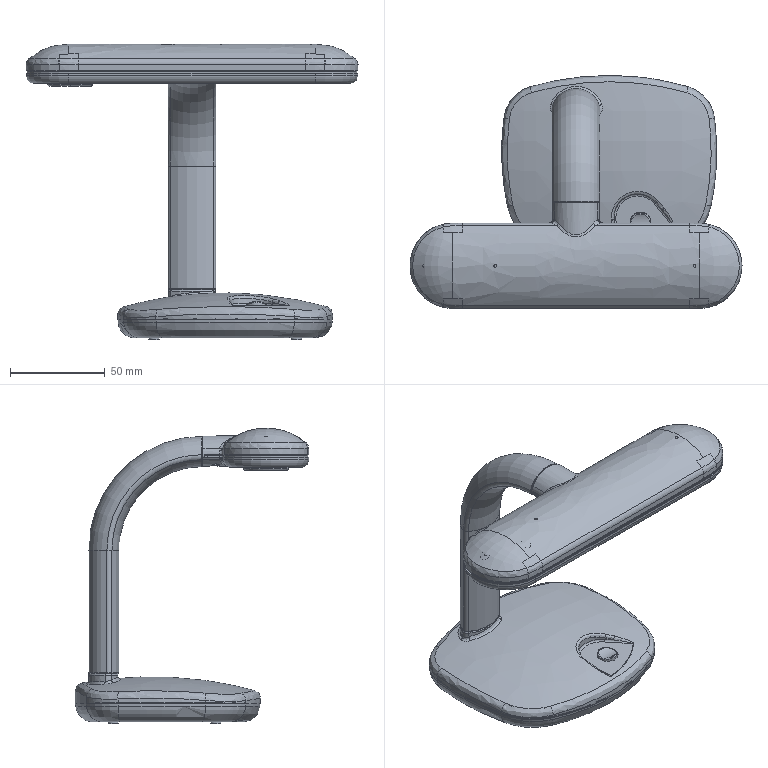Assembly | NX | mm | 9 component files | 9 solids | 848 faces | box 175 x 123.02 x 155.8 mm | volume 111281 mm3 | plane 324 | cylinder 252 | spline 133 | torus 67 | cone 66 | sphere 6 | commonest cylinder face diameters 1.5 x31 2 x25 5 x20 3 x20 1 x19 4 x18 6 x10 15 x8
Bill of materials:
unnamed part 1 | 1 |  | Flat rectangular plate with rounded corners and two through-holes, one near each end. Two rectangular tabs stick out from one long edge, leaving a notch between them.
unnamed part 2 | 1 |  | Flanged base with a short, slightly tapered cylindrical boss on top. The boss's top face is curved like a saddle. The flange has two lugs, each with a through-hole.
unnamed part 3 | 1 |  | Bent tubular body with a roughly 90-degree curve. It has a long straight leg ending in a smaller-diameter stepped end. A bore opens at the curved end.
unnamed part 4 | 1 |  | Elongated, pill-shaped low-profile body with a domed top. A short cylindrical stub sticks out sideways from the middle of one long side.
unnamed part 5 | 1 |  | Shallow, obround tray-like base with a perimeter rim. A raised rectangular block with one rounded end sits on the floor, small pins or bosses stand up from it, and a small bracket on one long side carries two holes.
unnamed part 6 | 1 |  | Rounded, squarish cover-like body with a gently domed top. It has two recessed pockets with through-holes: a small teardrop-shaped raised boss and a larger pocket shaped roughly like a sector.
unnamed part 7 | 1 |  | Bracket with a hexagonal outer profile and a rectangular through-opening. A flat mounting flange with two holed lugs extends from opposite sides, and there are also small holes in the side walls.
unnamed part 8 | 1 |  | Shallow open shell with a rounded-square outline and a thin perimeter wall. Inside are several cylindrical standoffs, a few small low bosses, and a grid of parallel slots.
unnamed part 9 | 1 |  | Long U-shaped tube with two parallel straight legs joined by a rounded bend. A collar and a small rectangular block with protruding thin pins sit at the open end.
Mates:
1. touch align | jiazhongkuai 1 | xiadizuo 1
2. touch align | jiazhongkuai 1 | xiadizuo 1
3. touch align | shangdizuo 1 | xiadizuo 1
4. touch align | shangdizuo 1 | xiadizuo 1
5. touch align | shangdizuo 1 | xiadizuo 1
6. touch align | anniu 1 | shangdizuo 1
7. touch align | anniu 1 | shangdizuo 1
8. touch align | shangdizuo 1 | anniu 1
9. fix | xiadizuo 1 component
10. distance | shangdizuo 1 | xiadizuo 1
11. fix | shangdengke 1 component
12. distance | shangdengke 1 | xiadengke 1
13. touch align | dizuozhuangpei 1 face | zhichengjia 1 face
14. touch align | zhichengjia 1 face | dizuozhuangpei 1 face
15. touch align | dengkezhuangpei 1 face | zhichengjia 1 face
16. touch align | dengkezhuangpei 1 face | zhichengjia 1 face
17. parallel | dengkezhuangpei 1 face | dizuozhuangpei 1 face
18. fix | dizuozhuangpei 1 component